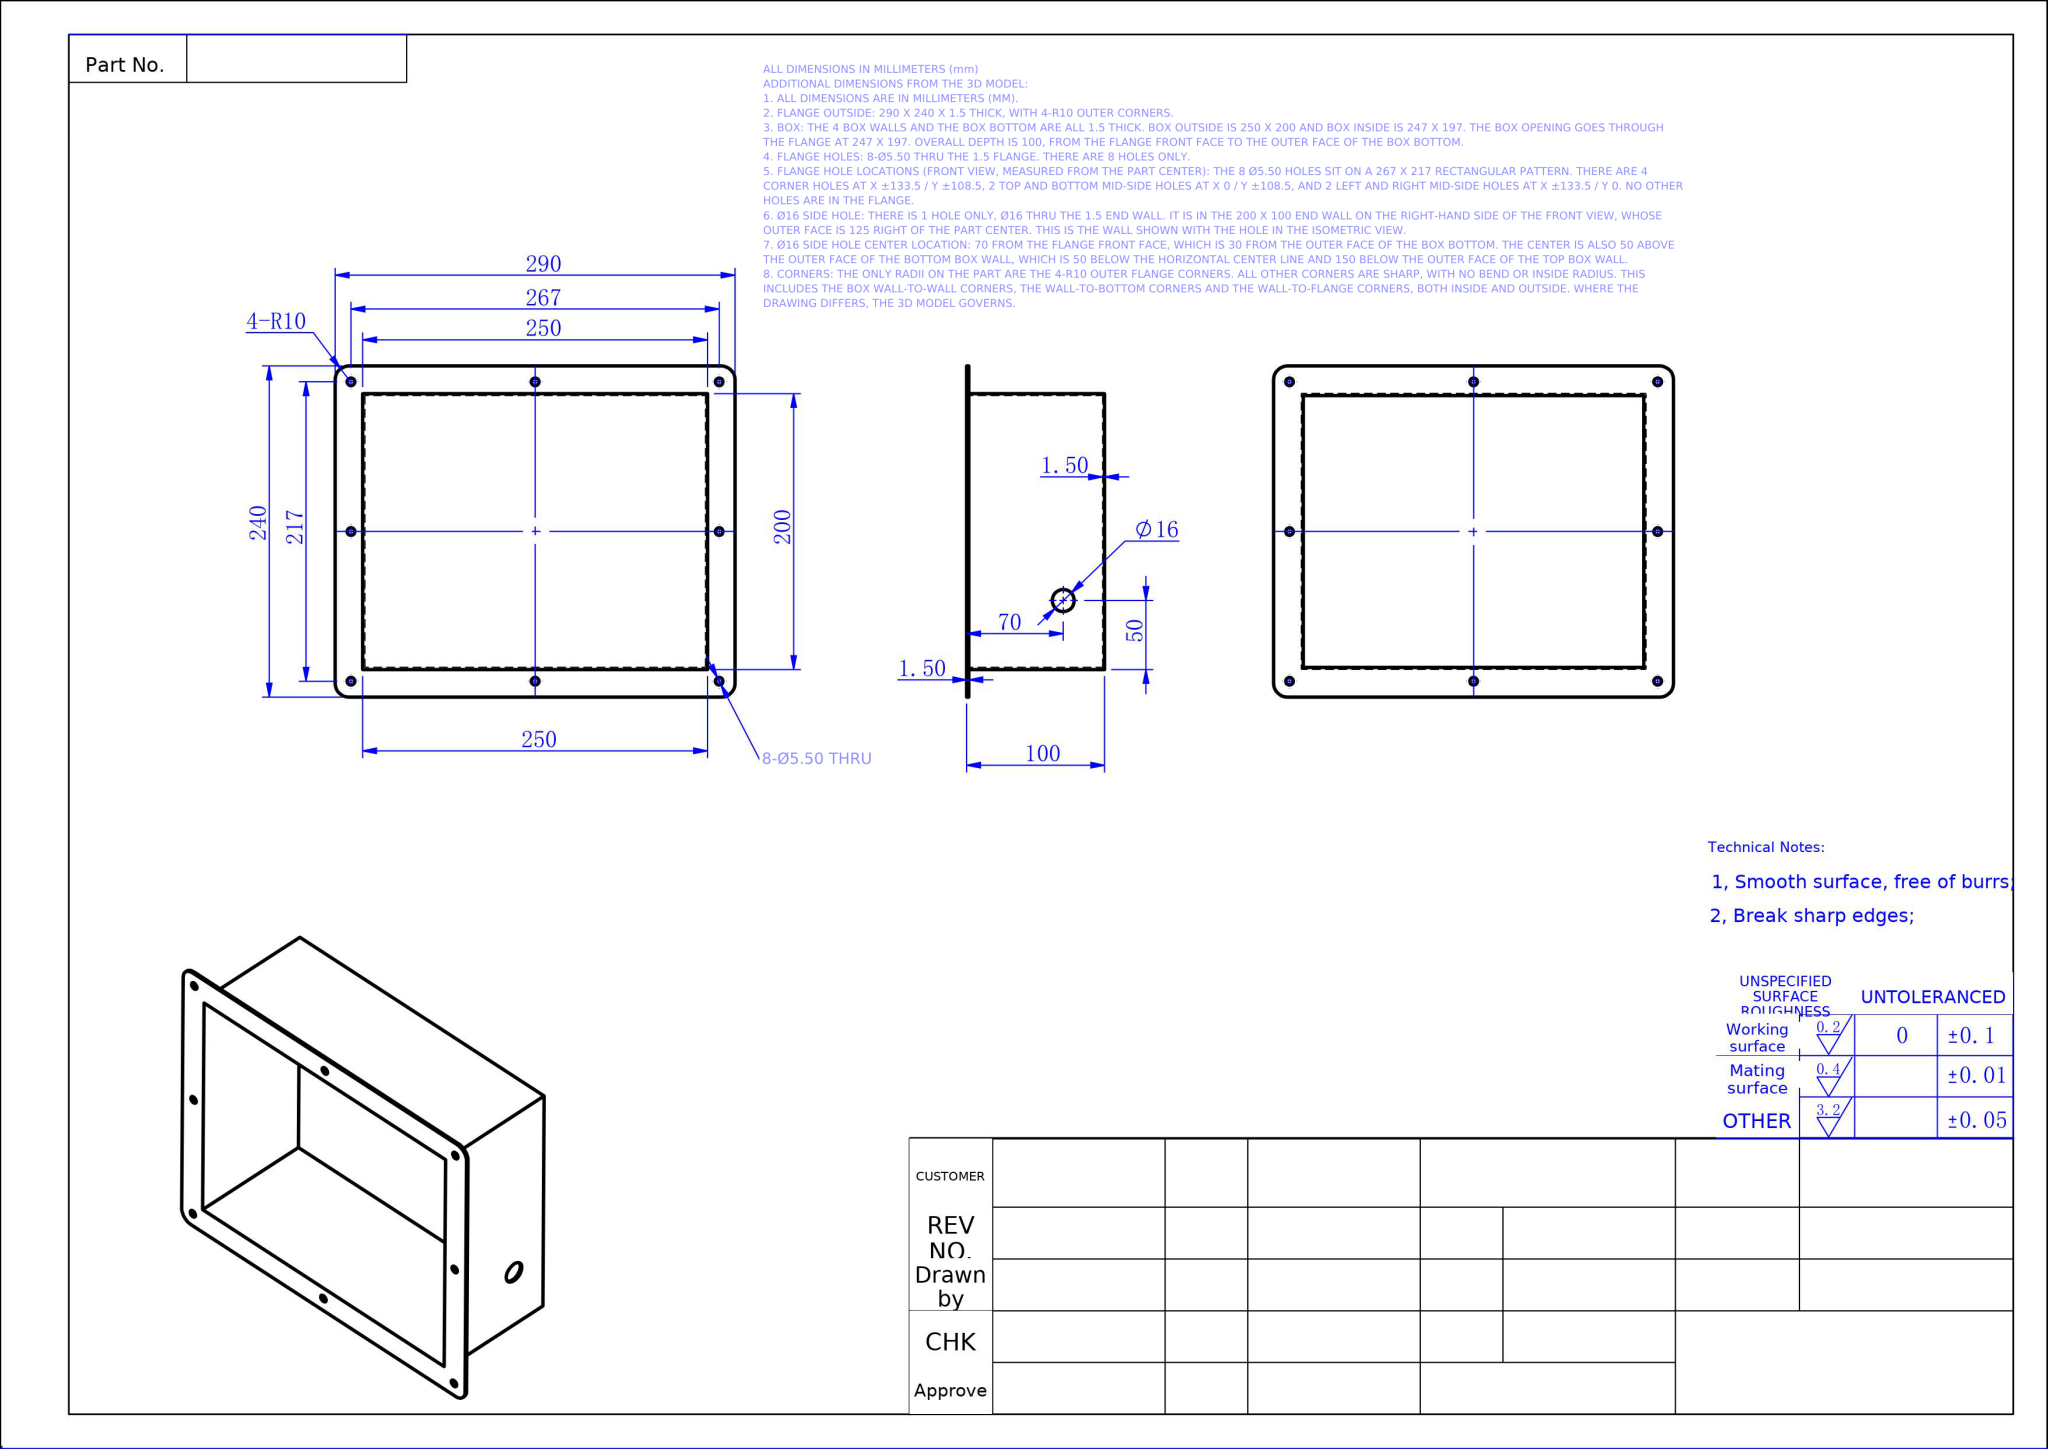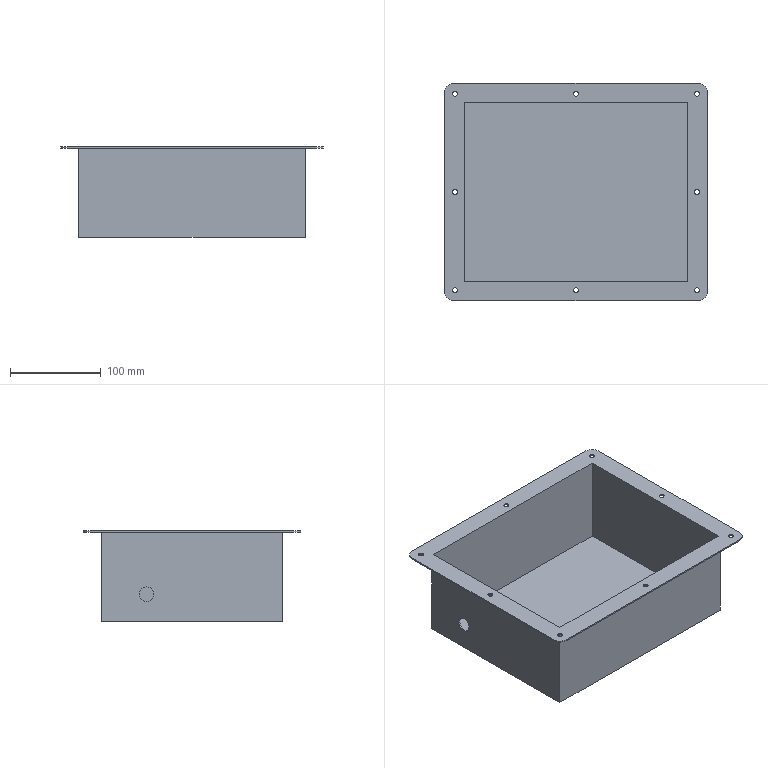Part | NX | mm | Flanged Rectangular Enclosure Tray | 1 solid | 38 faces | box 290 x 240 x 100 mm | volume 235773 mm3 | cylinder 22 | plane 16 | commonest cylinder face diameters 5.5 x16 20 x4 16 x2